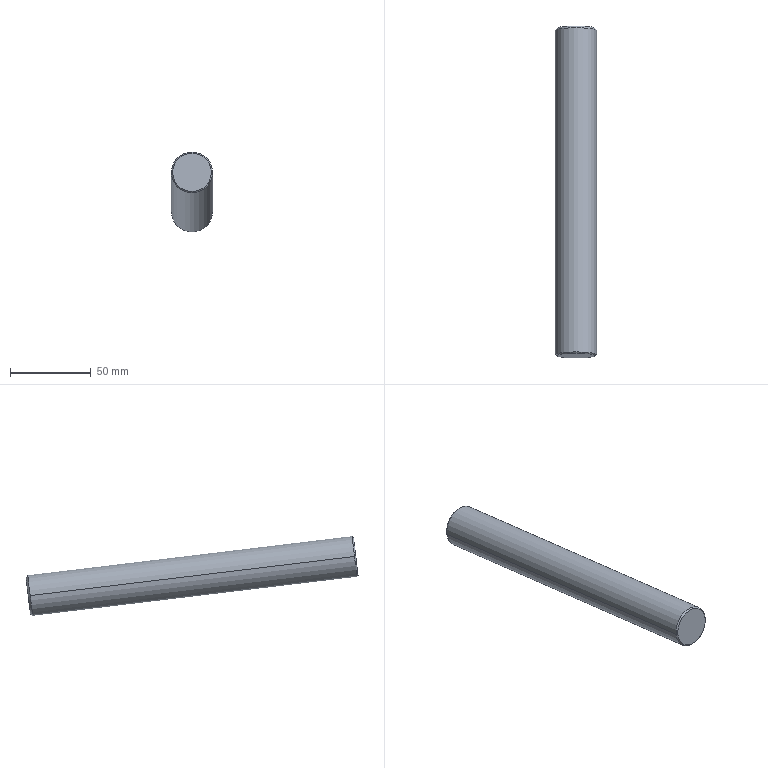Component | SolidWorks | DNR-71M20100BBEF2xx-A_500997-1_DNR-71M20100BBEF2xx-A_500996-2 | 1 solid | 8 faces | box 25.4 x 205.04 x 49.34 mm | volume 103135 mm3 | cone 4 | cylinder 2 | plane 2 | commonest cylinder face diameters 25.4 x2
STEP:
#1=COLOUR_RGB('',0.7922,0.8196,0.9333);
#2=FILL_AREA_STYLE_COLOUR('',#1);
#3=FILL_AREA_STYLE('',(#2));
#4=SURFACE_STYLE_FILL_AREA(#3);
#5=SURFACE_SIDE_STYLE('',(#4));
#6=SURFACE_STYLE_USAGE(.BOTH.,#5);
#7=PRESENTATION_STYLE_ASSIGNMENT((#6));
#8=CARTESIAN_POINT('',(11.425,4.861,5.4));
#9=VERTEX_POINT('',#8);
#10=CARTESIAN_POINT('',(12.325,4.861,5.4));
#11=VERTEX_POINT('',#10);
#12=CARTESIAN_POINT('',(11.875,4.861,5.4));
#13=DIRECTION('',(-0.,0.9928,-0.1196));
#14=DIRECTION('',(1.,0.,0.));
#15=AXIS2_PLACEMENT_3D('',#12,#13,#14);
#16=CIRCLE('',#15,0.45);
#17=EDGE_CURVE('',#9,#11,#16,.T.);
#18=ORIENTED_EDGE('',*,*,#17,.F.);
#19=CARTESIAN_POINT('',(11.375,4.811,5.406));
#20=VERTEX_POINT('',#19);
#21=CARTESIAN_POINT('',(11.425,4.861,5.4));
#22=DIRECTION('',(-0.7071,-0.702,0.08458));
#23=VECTOR('',#22,39.37);
#24=LINE('',#21,#23);
#25=EDGE_CURVE('',#9,#20,#24,.T.);
#26=ORIENTED_EDGE('',*,*,#25,.T.);
#27=CARTESIAN_POINT('',(12.375,4.811,5.406));
#28=VERTEX_POINT('',#27);
#29=CARTESIAN_POINT('',(11.875,4.811,5.406));
#30=DIRECTION('',(0.,-0.9928,0.1196));
#31=DIRECTION('',(1.,0.,0.));
#32=AXIS2_PLACEMENT_3D('',#29,#30,#31);
#33=CIRCLE('',#32,0.5);
#34=EDGE_CURVE('',#28,#20,#33,.T.);
#35=ORIENTED_EDGE('',*,*,#34,.F.);
#36=CARTESIAN_POINT('',(12.325,4.861,5.4));
#37=DIRECTION('',(0.7071,-0.702,0.08458));
#38=VECTOR('',#37,39.37);
#39=LINE('',#36,#38);
#40=EDGE_CURVE('',#11,#28,#39,.T.);
#41=ORIENTED_EDGE('',*,*,#40,.F.);
#42=EDGE_LOOP('',(#18,#26,#35,#41));
#43=FACE_OUTER_BOUND('',#42,.T.);
#44=CARTESIAN_POINT('',(11.875,4.861,5.4));
#45=DIRECTION('',(0.,-0.9928,0.1196));
#46=DIRECTION('',(1.,0.,0.));
#47=AXIS2_PLACEMENT_3D('',#44,#45,#46);
#48=CONICAL_SURFACE('',#47,0.45,0.7854);
#49=ADVANCED_FACE('',(#43),#48,.T.);
#50=CARTESIAN_POINT('',(12.345,-3.102,6.359));
#51=VERTEX_POINT('',#50);
#52=CARTESIAN_POINT('',(11.405,-3.102,6.359));
#53=VERTEX_POINT('',#52);
#54=CARTESIAN_POINT('',(11.875,-3.102,6.359));
#55=DIRECTION('',(0.,-0.9928,0.1196));
#56=DIRECTION('',(-1.,0.,0.));
#57=AXIS2_PLACEMENT_3D('',#54,#55,#56);
#58=CIRCLE('',#57,0.47);
#59=EDGE_CURVE('',#51,#53,#58,.T.);
#60=ORIENTED_EDGE('',*,*,#59,.F.);
#61=CARTESIAN_POINT('',(12.375,-3.072,6.356));
#62=VERTEX_POINT('',#61);
#63=CARTESIAN_POINT('',(12.375,-3.072,6.356));
#64=DIRECTION('',(0.7071,0.702,-0.08458));
#65=VECTOR('',#64,39.37);
#66=LINE('',#63,#65);
#67=EDGE_CURVE('',#51,#62,#66,.T.);
#68=ORIENTED_EDGE('',*,*,#67,.T.);
#69=CARTESIAN_POINT('',(11.375,-3.072,6.356));
#70=VERTEX_POINT('',#69);
#71=CARTESIAN_POINT('',(11.875,-3.072,6.356));
#72=DIRECTION('',(-0.,0.9928,-0.1196));
#73=DIRECTION('',(-1.,0.,0.));
#74=AXIS2_PLACEMENT_3D('',#71,#72,#73);
#75=CIRCLE('',#74,0.5);
#76=EDGE_CURVE('',#70,#62,#75,.T.);
#77=ORIENTED_EDGE('',*,*,#76,.F.);
#78=CARTESIAN_POINT('',(11.375,-3.072,6.356));
#79=DIRECTION('',(-0.7071,0.702,-0.08458));
#80=VECTOR('',#79,39.37);
#81=LINE('',#78,#80);
#82=EDGE_CURVE('',#53,#70,#81,.T.);
#83=ORIENTED_EDGE('',*,*,#82,.F.);
#84=EDGE_LOOP('',(#60,#68,#77,#83));
#85=FACE_OUTER_BOUND('',#84,.T.);
#86=CARTESIAN_POINT('',(11.875,-3.072,6.356));
#87=DIRECTION('',(-0.,0.9928,-0.1196));
#88=DIRECTION('',(-1.,0.,0.));
#89=AXIS2_PLACEMENT_3D('',#86,#87,#88);
#90=CONICAL_SURFACE('',#89,0.5,0.7854);
#91=ADVANCED_FACE('',(#85),#90,.T.);
#92=ORIENTED_EDGE('',*,*,#76,.T.);
#93=CARTESIAN_POINT('',(12.375,4.861,5.4));
#94=DIRECTION('',(-0.,0.9928,-0.1196));
#95=VECTOR('',#94,39.37);
#96=LINE('',#93,#95);
#97=EDGE_CURVE('',#62,#28,#96,.T.);
#98=ORIENTED_EDGE('',*,*,#97,.T.);
#99=ORIENTED_EDGE('',*,*,#34,.T.);
#100=CARTESIAN_POINT('',(11.375,4.861,5.4));
#101=DIRECTION('',(-0.,0.9928,-0.1196));
#102=VECTOR('',#101,39.37);
#103=LINE('',#100,#102);
#104=EDGE_CURVE('',#70,#20,#103,.T.);
#105=ORIENTED_EDGE('',*,*,#104,.F.);
#106=EDGE_LOOP('',(#92,#98,#99,#105));
#107=FACE_OUTER_BOUND('',#106,.T.);
#108=CARTESIAN_POINT('',(11.875,4.861,5.4));
#109=DIRECTION('',(-0.,0.9928,-0.1196));
#110=DIRECTION('',(-1.,0.,0.));
#111=AXIS2_PLACEMENT_3D('',#108,#109,#110);
#112=CYLINDRICAL_SURFACE('',#111,0.5);
#113=ADVANCED_FACE('',(#107),#112,.T.);
#114=CARTESIAN_POINT('',(11.875,4.861,5.4));
#115=DIRECTION('',(-0.,0.9928,-0.1196));
#116=DIRECTION('',(1.,0.,0.));
#117=AXIS2_PLACEMENT_3D('',#114,#115,#116);
#118=CIRCLE('',#117,0.45);
#119=EDGE_CURVE('',#11,#9,#118,.T.);
#120=ORIENTED_EDGE('',*,*,#119,.T.);
#121=ORIENTED_EDGE('',*,*,#17,.T.);
#122=EDGE_LOOP('',(#120,#121));
#123=FACE_OUTER_BOUND('',#122,.T.);
#124=CARTESIAN_POINT('',(11.875,4.861,5.4));
#125=DIRECTION('',(0.,-0.9928,0.1196));
#126=DIRECTION('',(1.,-0.,-0.));
#127=AXIS2_PLACEMENT_3D('',#124,#125,#126);
#128=PLANE('',#127);
#129=ADVANCED_FACE('',(#123),#128,.F.);
#130=ORIENTED_EDGE('',*,*,#97,.F.);
#131=CARTESIAN_POINT('',(11.875,-3.072,6.356));
#132=DIRECTION('',(-0.,0.9928,-0.1196));
#133=DIRECTION('',(-1.,0.,0.));
#134=AXIS2_PLACEMENT_3D('',#131,#132,#133);
#135=CIRCLE('',#134,0.5);
#136=EDGE_CURVE('',#62,#70,#135,.T.);
#137=ORIENTED_EDGE('',*,*,#136,.T.);
#138=ORIENTED_EDGE('',*,*,#104,.T.);
#139=CARTESIAN_POINT('',(11.875,4.811,5.406));
#140=DIRECTION('',(0.,-0.9928,0.1196));
#141=DIRECTION('',(1.,0.,0.));
#142=AXIS2_PLACEMENT_3D('',#139,#140,#141);
#143=CIRCLE('',#142,0.5);
#144=EDGE_CURVE('',#20,#28,#143,.T.);
#145=ORIENTED_EDGE('',*,*,#144,.T.);
#146=EDGE_LOOP('',(#130,#137,#138,#145));
#147=FACE_OUTER_BOUND('',#146,.T.);
#148=CARTESIAN_POINT('',(11.875,4.861,5.4));
#149=DIRECTION('',(-0.,0.9928,-0.1196));
#150=DIRECTION('',(-1.,0.,0.));
#151=AXIS2_PLACEMENT_3D('',#148,#149,#150);
#152=CYLINDRICAL_SURFACE('',#151,0.5);
#153=ADVANCED_FACE('',(#147),#152,.T.);
#154=CARTESIAN_POINT('',(11.875,-3.102,6.359));
#155=DIRECTION('',(0.,-0.9928,0.1196));
#156=DIRECTION('',(-1.,0.,0.));
#157=AXIS2_PLACEMENT_3D('',#154,#155,#156);
#158=CIRCLE('',#157,0.47);
#159=EDGE_CURVE('',#53,#51,#158,.T.);
#160=ORIENTED_EDGE('',*,*,#159,.T.);
#161=ORIENTED_EDGE('',*,*,#59,.T.);
#162=EDGE_LOOP('',(#160,#161));
#163=FACE_OUTER_BOUND('',#162,.T.);
#164=CARTESIAN_POINT('',(11.875,-3.102,6.359));
#165=DIRECTION('',(-0.,0.9928,-0.1196));
#166=DIRECTION('',(-1.,0.,0.));
#167=AXIS2_PLACEMENT_3D('',#164,#165,#166);
#168=PLANE('',#167);
#169=ADVANCED_FACE('',(#163),#168,.F.);
#170=ORIENTED_EDGE('',*,*,#67,.F.);
#171=ORIENTED_EDGE('',*,*,#159,.F.);
#172=ORIENTED_EDGE('',*,*,#82,.T.);
#173=ORIENTED_EDGE('',*,*,#136,.F.);
#174=EDGE_LOOP('',(#170,#171,#172,#173));
#175=FACE_OUTER_BOUND('',#174,.T.);
#176=CARTESIAN_POINT('',(11.875,-3.072,6.356));
#177=DIRECTION('',(-0.,0.9928,-0.1196));
#178=DIRECTION('',(-1.,0.,0.));
#179=AXIS2_PLACEMENT_3D('',#176,#177,#178);
#180=CONICAL_SURFACE('',#179,0.5,0.7854);
#181=ADVANCED_FACE('',(#175),#180,.T.);
#182=ORIENTED_EDGE('',*,*,#25,.F.);
#183=ORIENTED_EDGE('',*,*,#119,.F.);
#184=ORIENTED_EDGE('',*,*,#40,.T.);
#185=ORIENTED_EDGE('',*,*,#144,.F.);
#186=EDGE_LOOP('',(#182,#183,#184,#185));
#187=FACE_OUTER_BOUND('',#186,.T.);
#188=CARTESIAN_POINT('',(11.875,4.861,5.4));
#189=DIRECTION('',(0.,-0.9928,0.1196));
#190=DIRECTION('',(1.,0.,0.));
#191=AXIS2_PLACEMENT_3D('',#188,#189,#190);
#192=CONICAL_SURFACE('',#191,0.45,0.7854);
#193=ADVANCED_FACE('',(#187),#192,.T.);
#194=CLOSED_SHELL('',(#49,#91,#113,#129,#153,#169,#181,#193));
#195=MANIFOLD_SOLID_BREP('',#194);
#196=STYLED_ITEM('',(#7),#195);
#197=PRESENTATION_LAYER_ASSIGNMENT('','',(#196));
#198=(LENGTH_UNIT()NAMED_UNIT(*)SI_UNIT($,.METRE.));
#199=LENGTH_MEASURE_WITH_UNIT(LENGTH_MEASURE(0.0254),#198);
#200=DIMENSIONAL_EXPONENTS(1.,0.,0.,0.,0.,0.,0.);
#201=(CONVERSION_BASED_UNIT('',#199)LENGTH_UNIT()NAMED_UNIT(#200));
#202=UNCERTAINTY_MEASURE_WITH_UNIT(LENGTH_MEASURE(0.00001),#201,'','');
#203=(NAMED_UNIT(*)PLANE_ANGLE_UNIT()SI_UNIT($,.RADIAN.));
#204=(NAMED_UNIT(*)SI_UNIT($,.STERADIAN.)SOLID_ANGLE_UNIT());
#205=(GEOMETRIC_REPRESENTATION_CONTEXT(3)GLOBAL_UNCERTAINTY_ASSIGNED_CONTEXT((#202))GLOBAL_UNIT_ASSIGNED_CONTEXT((#201,#203,#204))REPRESENTATION_CONTEXT('',''));
#206=MECHANICAL_DESIGN_GEOMETRIC_PRESENTATION_REPRESENTATION('',(#196),#205);
#207=CARTESIAN_POINT('',(0.,0.,0.));
#208=DIRECTION('',(0.,0.,1.));
#209=DIRECTION('',(1.,0.,0.));
#210=AXIS2_PLACEMENT_3D('',#207,#208,#209);
#211=(LENGTH_UNIT()NAMED_UNIT(*)SI_UNIT($,.METRE.));
#212=LENGTH_MEASURE_WITH_UNIT(LENGTH_MEASURE(0.0254),#211);
#213=DIMENSIONAL_EXPONENTS(1.,0.,0.,0.,0.,0.,0.);
#214=(CONVERSION_BASED_UNIT('',#212)LENGTH_UNIT()NAMED_UNIT(#213));
#215=UNCERTAINTY_MEASURE_WITH_UNIT(LENGTH_MEASURE(0.00001),#214,'','');
#216=(NAMED_UNIT(*)PLANE_ANGLE_UNIT()SI_UNIT($,.RADIAN.));
#217=(NAMED_UNIT(*)SI_UNIT($,.STERADIAN.)SOLID_ANGLE_UNIT());
#218=(GEOMETRIC_REPRESENTATION_CONTEXT(3)GLOBAL_UNCERTAINTY_ASSIGNED_CONTEXT((#215))GLOBAL_UNIT_ASSIGNED_CONTEXT((#214,#216,#217))REPRESENTATION_CONTEXT('',''));
#219=ADVANCED_BREP_SHAPE_REPRESENTATION('',(#195,#210),#218);